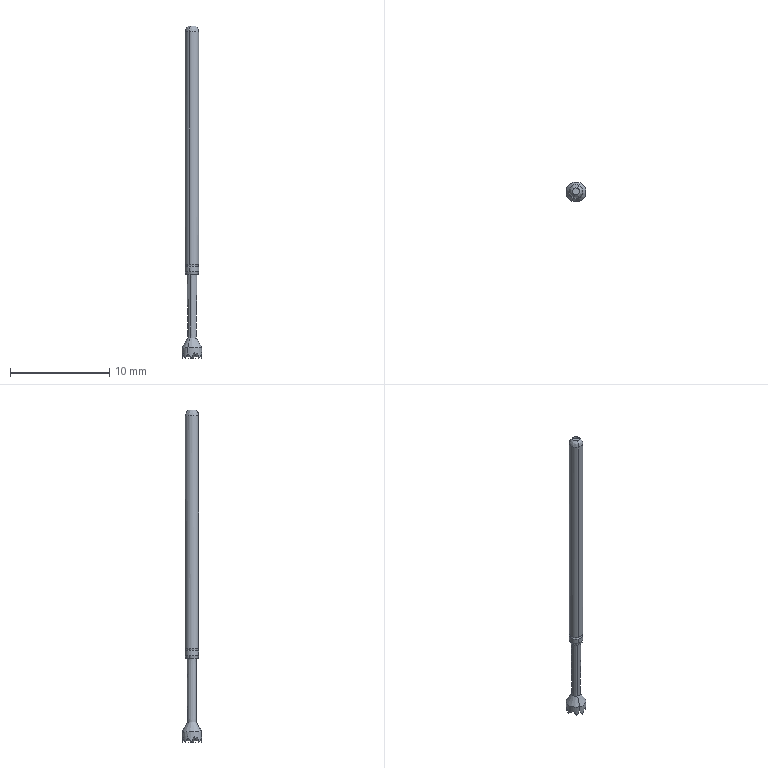Component | SolidWorks | 170423A4-GKS100-1_170423A4-GKS-100_306_200-1 | 1 solid | 152 faces | box 2 x 2 x 33.4 mm | volume 44 mm3 | spline 64 | plane 58 | cone 22 | cylinder 8 | commonest cylinder face diameters 1.366 x4 0.7 x2 2 x2